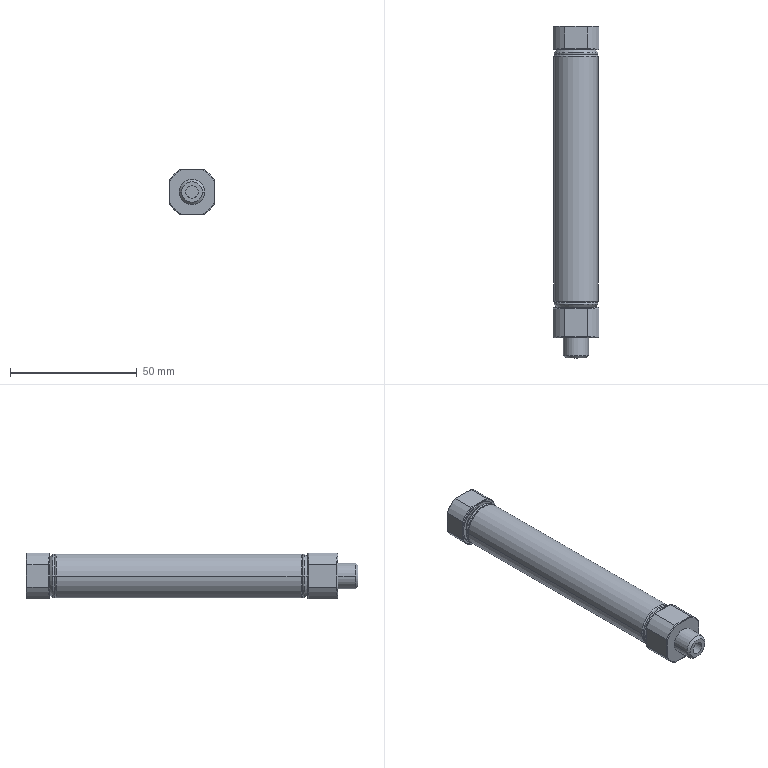Component | SolidWorks | PB_16x75_S_U_FA_M_2_0-1_16PB75UBody-1 | 1 solid | 110 faces | box 18 x 131 x 18 mm | volume 12401 mm3 | plane 48 | cone 30 | cylinder 24 | torus 8 | commonest cylinder face diameters 20 x8 4.134 x4 17.8 x4 16 x2 5 x2 17.4 x2 10 x2
build123d program:
from build123d import *

# Parameters (mm, degrees)
BOSS_EXTRUDE1_DEPTH     = 11.8
BOSS_EXTRUDE2_DEPTH     = 9.2
CUT_EXTRUDE1_DEPTH      = 9
CUT_EXTRUDE1_DEPTH_BACK = 9
CUT_EXTRUDE2_DEPTH      = 9
CUT_EXTRUDE2_DEPTH_BACK = 9
CUT_EXTRUDE3_DEPTH      = 9
CUT_EXTRUDE3_DEPTH_BACK = 9
CUT_EXTRUDE4_DEPTH      = 9
CUT_EXTRUDE4_DEPTH_BACK = 9
CUT_EXTRUDE5_DEPTH      = 9
CUT_EXTRUDE5_DEPTH_BACK = 9
CUT_EXTRUDE6_DEPTH      = 9
CUT_EXTRUDE6_DEPTH_BACK = 9
CUT_EXTRUDE7_DEPTH      = 9
CUT_EXTRUDE7_DEPTH_BACK = 9
CUT_EXTRUDE8_DEPTH      = 9
CUT_EXTRUDE8_DEPTH_BACK = 9


with BuildPart() as part:
    # Sketch1 → Revolve1 (revolve)
    with BuildSketch(Plane.XY, mode=Mode.PRIVATE) as revolve1_sk:
        Polygon((0, 0), (0, 4.08), (0.92, 5), (8, 5), (8, 0), align=None)
    revolve(revolve1_sk.sketch.rotate(Axis((8, 0, 0), (-1, 0, 0)), 270), axis=Axis((8, 0, 0), (-1, 0, 0)))

    # Sketch2 → Boss-Extrude1 (add)
    with BuildSketch(Plane(origin=(8, 0, 0), x_dir=(0, 0, -1), z_dir=(1, 0, 0))):
        with BuildLine():
            Line((-9, 7.937), (-9, -7.937))
            ThreePointArc((-9, -7.937), (-8.485, -8.485), (-7.937, -9))
            Line((-7.937, -9), (7.937, -9))
            ThreePointArc((7.937, -9), (8.485, -8.485), (9, -7.937))
            Line((9, -7.937), (9, 7.937))
            ThreePointArc((9, 7.937), (8.485, 8.485), (7.937, 9))
            Line((7.937, 9), (-7.937, 9))
            ThreePointArc((-7.937, 9), (-8.485, 8.485), (-9, 7.937))
        make_face()
    extrude(amount=BOSS_EXTRUDE1_DEPTH)

    # Sketch3 → Cut-Revolve1 (revolve, cut)
    with BuildSketch(Plane.XY):
        Polygon((8, 20), (8, 9.7), (8.3, 10), (19.5, 10), (19.8, 9.7), (19.8, 20), align=None)
    revolve(axis=Axis((19.8, 0, 0), (-1, 0, 0)), mode=Mode.SUBTRACT)

    # Sketch4 → Revolve2 (revolve)
    with BuildSketch(Plane.XY, mode=Mode.PRIVATE) as revolve2_sk:
        with BuildLine():
            Line((19.8, 0), (19.8, 8.9))
            Line((19.8, 8.9), (19.95, 8.9))
            Line((19.95, 8.9), (19.95, 7.62))
            Line((19.95, 7.62), (21.038, 8.533))
            ThreePointArc((21.038, 8.533), (21.403, 8.648), (21.742, 8.471))
            Line((21.742, 8.471), (21.97, 8.2))
            ThreePointArc((21.97, 8.2), (22.157, 8.506), (22.46, 8.7))
            Line((22.46, 8.7), (119.14, 8.7))
            ThreePointArc((119.14, 8.7), (119.443, 8.506), (119.63, 8.2))
            Line((119.63, 8.2), (119.858, 8.471))
            ThreePointArc((119.858, 8.471), (120.197, 8.648), (120.562, 8.533))
            Line((120.562, 8.533), (121.65, 7.62))
            Line((121.65, 7.62), (121.65, 8.9))
            Line((121.65, 8.9), (121.8, 8.9))
            Line((121.8, 8.9), (121.8, 0))
            Line((121.8, 0), (19.8, 0))
        make_face()
    revolve(revolve2_sk.sketch.rotate(Axis((121.8, 0, 0), (-1, 0, 0)), 270), axis=Axis((121.8, 0, 0), (-1, 0, 0)))

    # Sketch5 → Boss-Extrude2 (add)
    with BuildSketch(Plane(origin=(121.8, 0, 0), x_dir=(0, 0, -1), z_dir=(1, 0, 0))):
        with BuildLine():
            Line((-9, 6.325), (-9, -6.325))
            ThreePointArc((-9, -6.325), (-7.778, -7.778), (-6.325, -9))
            Line((-6.325, -9), (6.325, -9))
            ThreePointArc((6.325, -9), (7.778, -7.778), (9, -6.325))
            Line((9, -6.325), (9, 6.325))
            ThreePointArc((9, 6.325), (7.778, 7.778), (6.325, 9))
            Line((6.325, 9), (-6.325, 9))
            ThreePointArc((-6.325, 9), (-7.778, 7.778), (-9, 6.325))
        make_face()
    extrude(amount=BOSS_EXTRUDE2_DEPTH)

    # Sketch6 → Cut-Revolve2 (revolve, cut)
    with BuildSketch(Plane.XY):
        Polygon((121.8, 20), (121.8, 9.7), (122.1, 10), (130.7, 10), (131, 9.7), (131, 20), align=None)
    revolve(axis=Axis((131, 0, 0), (-1, 0, 0)), mode=Mode.SUBTRACT)

    # Sketch7 → Cut-Revolve3 (revolve, cut)
    with BuildSketch(Plane.XY, mode=Mode.PRIVATE) as cut_revolve3_sk:
        Polygon((15.5, 9), (18, 9), (17.567, 8.567), (17.567, 0.9), (15.5, 0.9), align=None)
    revolve(cut_revolve3_sk.sketch.rotate(Axis((15.5, 0.9, 0), (0, 1, 0)), 270), axis=Axis((15.5, 0.9, 0), (0, 1, 0)), mode=Mode.SUBTRACT)

    # Sketch8 → Cut-Revolve4 (revolve, cut)
    with BuildSketch(Plane.XY, mode=Mode.PRIVATE) as cut_revolve4_sk:
        Polygon((126.2, 9), (128.7, 9), (128.267, 8.567), (128.267, 0.9), (126.2, 0.9), align=None)
    revolve(cut_revolve4_sk.sketch.rotate(Axis((126.2, 0.9, 0), (0, 1, 0)), 270), axis=Axis((126.2, 0.9, 0), (0, 1, 0)), mode=Mode.SUBTRACT)

    # Sketch9 → Cut-Revolve5 (revolve, cut)
    with BuildSketch(Plane.XY, mode=Mode.PRIVATE) as cut_revolve5_sk:
        Polygon((0, 0), (0, 2.5), (27.16, 2.5), (27.16, 8), (115.36, 8), (115.36, 0), align=None)
    revolve(cut_revolve5_sk.sketch.rotate(Axis((115.36, 0, 0), (-1, 0, 0)), 270), axis=Axis((115.36, 0, 0), (-1, 0, 0)), mode=Mode.SUBTRACT)

    # Sketch10 → Cut-Extrude1 (cut, two sides: drawn at the far end of the back side and taken through both)
    with BuildSketch(Plane.XY.offset(-CUT_EXTRUDE1_DEPTH_BACK)):
        Polygon((8, 8.7), (8.3, 9), (19.5, 9), (19.8, 8.7), (19.8, 10), (8, 10), align=None)
    extrude(amount=CUT_EXTRUDE1_DEPTH + CUT_EXTRUDE1_DEPTH_BACK, mode=Mode.SUBTRACT)

    # Sketch11 → Cut-Extrude2 (cut, two sides: drawn at the far end of the back side and taken through both)
    with BuildSketch(Plane.XY.offset(-CUT_EXTRUDE2_DEPTH_BACK)):
        Polygon((8, -8.7), (8, -10), (19.8, -10), (19.8, -8.7), (19.5, -9), (8.3, -9), align=None)
    extrude(amount=CUT_EXTRUDE2_DEPTH + CUT_EXTRUDE2_DEPTH_BACK, mode=Mode.SUBTRACT)

    # Sketch12 → Cut-Extrude3 (cut, two sides: drawn at the far end of the back side and taken through both)
    with BuildSketch(Plane(origin=(0, 0, 0), x_dir=(1, 0, 0), z_dir=(0, 1, 0)).offset(-CUT_EXTRUDE3_DEPTH_BACK)):
        Polygon((8, 8.7), (8.3, 9), (19.5, 9), (19.8, 8.7), (19.8, 10), (8, 10), align=None)
    extrude(amount=CUT_EXTRUDE3_DEPTH + CUT_EXTRUDE3_DEPTH_BACK, mode=Mode.SUBTRACT)

    # Sketch13 → Cut-Extrude4 (cut, two sides: drawn at the far end of the back side and taken through both)
    with BuildSketch(Plane(origin=(0, 0, 0), x_dir=(1, 0, 0), z_dir=(0, 1, 0)).offset(-CUT_EXTRUDE4_DEPTH_BACK)):
        Polygon((8, -8.7), (8, -10), (19.8, -10), (19.8, -8.7), (19.5, -9), (8.3, -9), align=None)
    extrude(amount=CUT_EXTRUDE4_DEPTH + CUT_EXTRUDE4_DEPTH_BACK, mode=Mode.SUBTRACT)

    # Sketch14 → Cut-Extrude5 (cut, two sides: drawn at the far end of the back side and taken through both)
    with BuildSketch(Plane.XY.offset(-CUT_EXTRUDE5_DEPTH_BACK)):
        Polygon((121.8, 8.7), (122.1, 9), (130.7, 9), (131, 8.7), (131, 10), (121.8, 10), align=None)
    extrude(amount=CUT_EXTRUDE5_DEPTH + CUT_EXTRUDE5_DEPTH_BACK, mode=Mode.SUBTRACT)

    # Sketch15 → Cut-Extrude6 (cut, two sides: drawn at the far end of the back side and taken through both)
    with BuildSketch(Plane.XY.offset(-CUT_EXTRUDE6_DEPTH_BACK)):
        Polygon((121.8, -8.7), (121.8, -10), (131, -10), (131, -8.7), (130.7, -9), (122.1, -9), align=None)
    extrude(amount=CUT_EXTRUDE6_DEPTH + CUT_EXTRUDE6_DEPTH_BACK, mode=Mode.SUBTRACT)

    # Sketch16 → Cut-Extrude7 (cut, two sides: drawn at the far end of the back side and taken through both)
    with BuildSketch(Plane(origin=(0, 0, 0), x_dir=(1, 0, 0), z_dir=(0, 1, 0)).offset(-CUT_EXTRUDE7_DEPTH_BACK)):
        Polygon((121.8, 8.7), (122.1, 9), (130.7, 9), (131, 8.7), (131, 10), (121.8, 10), align=None)
    extrude(amount=CUT_EXTRUDE7_DEPTH + CUT_EXTRUDE7_DEPTH_BACK, mode=Mode.SUBTRACT)

    # Sketch17 → Cut-Extrude8 (cut, two sides: drawn at the far end of the back side and taken through both)
    with BuildSketch(Plane(origin=(0, 0, 0), x_dir=(1, 0, 0), z_dir=(0, 1, 0)).offset(-CUT_EXTRUDE8_DEPTH_BACK)):
        Polygon((121.8, -8.7), (121.8, -10), (131, -10), (131, -8.7), (130.7, -9), (122.1, -9), align=None)
    extrude(amount=CUT_EXTRUDE8_DEPTH + CUT_EXTRUDE8_DEPTH_BACK, mode=Mode.SUBTRACT)


solid = part.part

# Placed as in the assembly
solid = solid.moved(Location((45, -230.5, 55), (-90, -90, 0)))